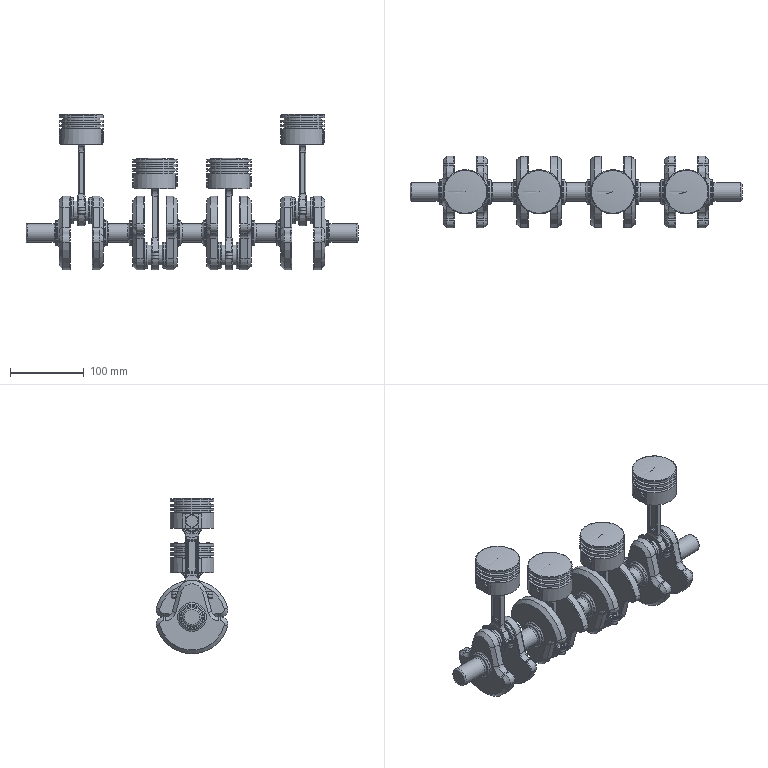Assembly | NX | mm | 13 component files | 17 solids | 1149 faces | box 450 x 97.46 x 211.04 mm | volume 1219595 mm3 | cylinder 345 | torus 286 | plane 270 | spline 148 | cone 100 | commonest cylinder face diameters 2 x80 20 x48 3 x32 40 x24 35 x20 10 x16 4 x16 24 x16
Bill of materials:
unnamed part 1 | 4 |  | Half-round (semicircular) strap or cap: a curved band of constant rectangular cross-section ending in two flat, round-ended tabs, each with one through-hole.
unnamed part 2 | 1 |  | Long multi-throw shaft resembling a crankshaft: coaxial cylindrical journals with plain cylindrical ends, plus several pairs of webs (disc-like plates) carrying offset cylindrical pins between them.
unnamed part 3 | 4 |  | Short cylindrical, piston-like body: a flat or slightly domed top, three circumferential grooves near the top, and two opposite circular bosses on the lower side wall.
unnamed part 4 | 4 |  | Rod-like link resembling a connecting rod: a round eye with a bore at one end, a straight beam with a recessed pocket, and at the other end a semicircular opening flanked by two flat tabs, each with a through-hole.
Mates:
1. touch align | Con_Rod 1 | Piston 1
2. distance | Con_Rod 1 | Piston 1
3. concentric | Con_CAP 1 | Con_Rod 1
4. concentric | Con_CAP 1 | Con_Rod 1
5. fix | crank 1 component
6. touch align | Sub_Assy 4 face | crank 1 face
7. distance | Sub_Assy 4 face | crank 1 face
8. distance | Sub_Assy 3 face | crank 1 face
9. touch align | Sub_Assy 3 face | crank 1 face
10. distance | Sub_Assy 2 face | crank 1 face
11. touch align | Sub_Assy 2 face | crank 1 face
12. touch align | Sub_Assy 1 face | crank 1 face
13. distance | Sub_Assy 1 face | crank 1 face